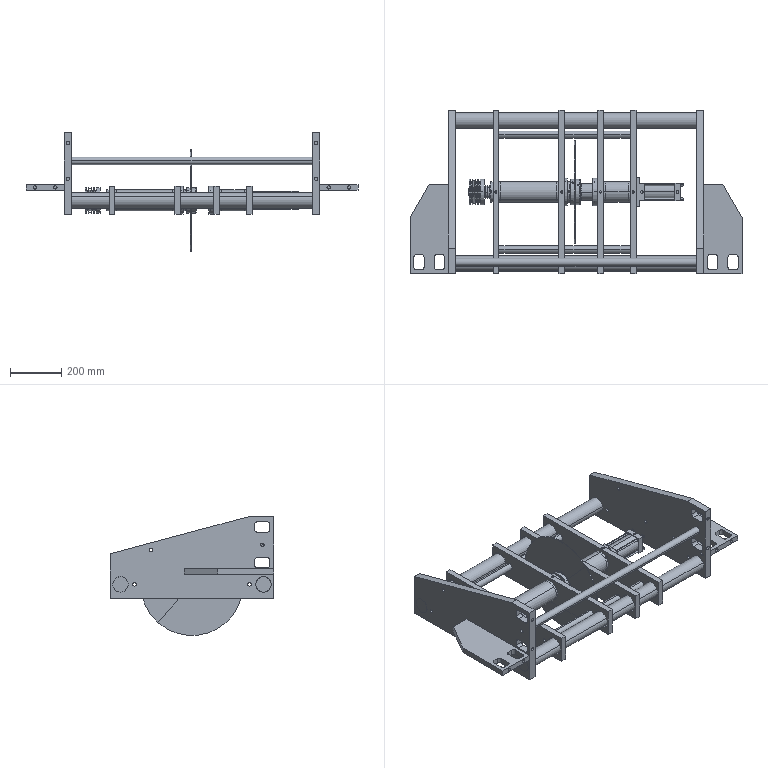Assembly | SolidWorks | mm | 50 component files | 156 solids | 2266 faces | box 1300 x 640 x 465 mm | volume 26290505 mm3 | cylinder 957 | plane 475 | sphere 364 | torus 242 | cone 228 | commonest cylinder face diameters 6.277 x72 7.03 x72 13 x64 8.017 x52 8.979 x52 20 x36 5 x34 9 x24
Bill of materials:
2-10-1WorkpieceAxisBearingHousing | 1 |  | Long hollow cylindrical tube with a wider circular flange at one end; the flange face has a large central bore, four larger through-holes and four smaller holes that look countersunk or chamfered, spaced around it.
2-10-2WorkpieceAxis | 1 |  | Long slender stepped cylindrical shaft with several diameter changes along its length; a coaxial hole with a cone-shaped bottom at one end and a small cross hole near that end.
2-10-3BearingSideCover | 2 |  | Flat circular ring-shaped plate with a large central bore, four evenly spaced through-holes near the outer edge, and a thin raised boss of smaller diameter on one face.
2-10-4Bushing | 1 |  | Thin-walled cylindrical sleeve or band with a short axial length compared to its diameter, and small chamfers on its edges.
2-10-5LockNut | 2 |  | Flat annular ring with four rectangular slots cut into its outer edge, evenly spaced; edges are chamfered.
2-10-6BearingShim | 1 |  | Thin flat annular ring (washer-like disk) with a plain round inner hole and outer edge.
2-10-7OilSealTC-40X52X7 | 2 | Rubber | Short cylindrical ring with a rectangular cross-section and an internal step or shoulder visible on one face.
2-10-8Bearing7007AC | 2 |  | Radial ball bearing-like assembly: concentric inner and outer rings with a single row of spherical balls between them, plus a thin ring-shaped element running between the balls.
2-10-9Bearing51107 | 1 |  | Axial thrust ball bearing-like assembly: two flat annular washers with a single row of balls held in a ring between them.
Flange1 | 1 |  | Thick flat circular disk with a central bore and two smaller through-holes on opposite sides; one radial hole in the outer edge; edges are chamfered.
4-12-10SplineConnectionAxisOilSealTC40X55X7 | 1 | Rubber | Cylindrical ring with a rectangular cross-section and an internal step or shoulder on one face, similar to the other stepped rings.
4-12-11TelescopicAxisOilSealTC64X80X12 | 1 | Rubber | Cylindrical ring with a fairly thin radial wall and a small internal step or groove near one face.
4-12-1ClampingTelescopicAxisHousing | 1 |  | Flanged hollow tube: a long thin-walled cylindrical sleeve with a round flange at one end that has four small holes.
4-12-2TelescopicAxis | 1 |  | Solid cylinder with a small central axial hole; looks like a thick-walled spacer or sleeve.
4-12-3ClampingAxis | 1 |  | Stepped cylindrical pin: a short larger-diameter head with a small cross hole, a raised collar, and a long, smaller-diameter shaft with a chamfered end.
4-12-4Bearing6005-2RZ | 3 |  | Ring assembly with concentric inner and outer rings and a circle of balls between them; its shape resembles a radial ball bearing.
4-12-551205Bearing | 1 |  | Axial stack of two flat annular rings with a ring of balls held between them; its shape resembles a thrust ball bearing.
4-12-6ClampingAxisBearingOuterPad | 1 |  | Short, plain, thin-walled cylindrical tube or sleeve.
4-12-7ClampingAxisBearingInnerPad | 1 |  | Plain cylindrical sleeve or bushing, with a thicker wall than the similar thin-walled tube in this set.
4-12-8ClampingAxis51205BearingShim | 1 |  | Thin flat annular ring, washer-like in shape.
4-12-9HeadlessSetScrew-D10 | 1 |  | Stepped solid round part: a smaller-diameter cylindrical spigot, a conical transition, and a larger-diameter cylindrical body with a chamfered end.
Crossbeam | 2 |  | Long, slender solid cylindrical rod with plain flat ends.
MainBracket | 2 |  | Flat plate with an irregular four-sided outline (one sloped edge), cut with two large round holes, two rounded-rectangle openings and several small holes.
SideReinforcementPlate | 2 |  | Thick flat plate with one angled corner and two rounded-rectangle through openings near one end; small holes drilled into its edge faces.
AxisHousingBracket | 4 |  | Long flat rectangular bar with three large round through-holes (one at the center, one near each end) and two small round through-holes, each just inboard of an end hole; a small hole also enters the long top edge at mid-length.
FeedingClampingCylinder | 1 |  | Cylinder-like body: a round barrel held between two square end blocks by four rods along its length, with hex nuts on the rod ends at one block. A stepped round shaft sticks out from the other end, which also has a rectangular flange with four corner holes. Each end block has a round hole in its top face.
FixedLengthRod | 1 |  | Long, slender round rod or tube with a small central hole at the end; in the end view the hole appears to have a cone-shaped, faceted bottom.
Flange2 | 1 |  | Thick ring or collar with a central through-bore, small chamfers on the outer edges, and one small radial hole in the outer cylindrical surface.
LocatingGuideBushing106 | 2 |  | Cylindrical tube or sleeve with a concentric through-bore, chamfered outer ends and chamfered bore entrances; its length is about four times its diameter.
LocatingGuideBushing130 | 2 |  | Cylindrical tube or sleeve with a concentric through-bore, chamfered outer ends and chamfered bore entrances; it is more slender than unnamed part.
LocatingGuideBushing156 | 2 |  | Long, slender cylindrical tube with a concentric through-bore, small chamfers on the outer ends and chamfered bore entrances; it is the most elongated of the similar sleeves.
Oil-impregnatedBushing | 2 |  | Thin-walled cylindrical ring or band whose width is a large fraction of its diameter, with plain inner and outer cylindrical surfaces and slight edge breaks.
SawBlade400 | 1 |  | Very thin flat circular disc with a small central hole and two smaller holes placed diagonally opposite each other near the center.
SawBladeDrivePulley | 1 |  | Multi-groove V-pulley (sheave) with four V-shaped grooves around its circumference, a wider plain cylindrical band on one side, and a central bore with a rectangular keyway.
Mates:
1. concentric | 4-12-12ClampingAxisAssembly-1/4-12-3ClampingAxis-1 face at (-152.809, -4.181, 0) dir (-1, 0, 0) r 16 | 2-10-10WorkpieceAxisAssembly-1/2-10-2WorkpieceAxis-1 face at (-157.809, -4.181, 0) dir (-1, 0, 0) r 16
2. concentric | 4-12-12ClampingAxisAssembly-1/4-12-1ClampingTelescopicAxisHousing-1 face at (-87.809, -4.181, 0) dir (-1, 0, 0) r 41 | AxisHousingBracket-1 face at (-67.809, -4.181, 0) dir (1, 0, 0) r 41
3. coincident | 4-12-12ClampingAxisAssembly-1/4-12-1ClampingTelescopicAxisHousing-1 face at (-67.809, 50.819, 0) dir (1, 0, 0) | AxisHousingBracket-1 face at (-67.809, -324.181, 55) dir (-1, 0, 0)
4. concentric | 4-12-12ClampingAxisAssembly-1/4-12-1ClampingTelescopicAxisHousing-1 face at (-87.809, 29.76, 33.941) dir (-1, 0, 0) r 3.3 | AxisHousingBracket-1 face at (-67.809, 29.76, 33.941) dir (-1, 0, 0) r 2.5
5. concentric | 2-10-10WorkpieceAxisAssembly-1/2-10-1WorkpieceAxisBearingHousing-1 face at (-187.809, -4.181, 0) dir (1, 0, 0) r 41 | AxisHousingBracket-2 face at (60.191, -4.181, 0) dir (1, 0, 0) r 41
6. concentric | AxisHousingBracket-1 face at (-67.809, 275.819, 0) dir (1, 0, 0) r 35 | AxisHousingBracket-2 face at (60.191, 275.819, 0) dir (1, 0, 0) r 35
7. coincident | 4-12-12ClampingAxisAssembly-1/4-12-1ClampingTelescopicAxisHousing-1 face at (82.191, 36.819, 0) dir (1, 0, 0) | AxisHousingBracket-2 face at (82.191, -324.181, 55) dir (1, 0, 0)
8. concentric | 2-10-10WorkpieceAxisAssembly-1/2-10-1WorkpieceAxisBearingHousing-1 face at (-187.809, -4.181, 0) dir (1, 0, 0) r 41 | AxisHousingBracket-3 face at (-197.809, -4.181, 0) dir (-1, 0, 0) r 41
9. coincident | 2-10-10WorkpieceAxisAssembly-1/2-10-1WorkpieceAxisBearingHousing-1 face at (-197.809, 36.556, 36.952) dir (-1, 0, 0) | AxisHousingBracket-3 face at (-197.809, 315.819, 55) dir (1, 0, 0)
10. coincident | AxisHousingBracket-1 face at (-67.809, 315.819, 55) dir (0, 0, 1) | AxisHousingBracket-3 face at (-197.809, -324.181, 55) dir (0, 0, 1)
11. concentric | 2-10-10WorkpieceAxisAssembly-1/2-10-1WorkpieceAxisBearingHousing-1 face at (-187.809, -4.181, 0) dir (1, 0, 0) r 41 | AxisHousingBracket-4 face at (-477.809, -4.181, 0) dir (1, 0, 0) r 41
12. parallel | AxisHousingBracket-3 face at (-197.809, -324.181, 55) dir (0, 0, 1) | AxisHousingBracket-4 face at (-477.809, 315.819, 55) dir (0, 0, 1)
13. coincident | 2-10-10WorkpieceAxisAssembly-1/2-10-3BearingSideCover-2 edge at (-477.809, -4.181, 0) dir (1, 0, 0) r 41 | AxisHousingBracket-4 face at (-477.809, -324.181, 55) dir (-1, 0, 0)
14. distance | AxisHousingBracket-1 face at (-67.809, -324.181, 55) dir (-1, 0, 0) | AxisHousingBracket-3 face at (-197.809, 315.819, 55) dir (1, 0, 0)
15. coincident | AxisHousingBracket-3 face at (-197.809, 315.819, 55) dir (1, 0, 0) | LocatingGuideBushing130-1 face at (-197.809, -229.181, 0) dir (-1, 0, 0)
16. concentric | AxisHousingBracket-3 face at (-219.809, -229.181, 0) dir (1, 0, 0) r 6.5 | LocatingGuideBushing130-1 face at (-67.809, -229.181, 0) dir (-1, 0, 0) r 14
17. coincident | AxisHousingBracket-3 face at (-197.809, 315.819, 55) dir (1, 0, 0) | LocatingGuideBushing130-2 face at (-197.809, 220.819, 0) dir (-1, 0, 0)
18. concentric | AxisHousingBracket-3 face at (-219.809, 220.819, 0) dir (1, 0, 0) r 6.5 | LocatingGuideBushing130-2 face at (-67.809, 220.819, 0) dir (-1, 0, 0) r 6.5
19. concentric | LocatingGuideBushing130-2 face at (-67.809, 220.819, 0) dir (-1, 0, 0) r 14 | LocatingGuideBushing106-1 face at (-45.809, 220.819, 0) dir (1, 0, 0) r 14
20. coincident | AxisHousingBracket-2 face at (60.191, -324.181, 55) dir (-1, 0, 0) | LocatingGuideBushing106-1 face at (60.191, 220.819, 0) dir (1, 0, 0)
21. concentric | AxisHousingBracket-3 face at (-219.809, 220.819, 0) dir (1, 0, 0) r 6.5 | LocatingGuideBushing156-1 face at (-219.809, 220.819, 0) dir (-1, 0, 0) r 14
22. coincident | AxisHousingBracket-3 face at (-219.809, 315.819, 55) dir (-1, 0, 0) | LocatingGuideBushing156-1 face at (-219.809, 220.819, 0) dir (1, 0, 0)
23. concentric | AxisHousingBracket-3 edge at (-219.809, -229.181, 0) dir (1, 0, 0) r 6.5 | LocatingGuideBushing156-2 face at (-219.809, -229.181, 0) dir (-1, 0, 0) r 14
24. coincident | AxisHousingBracket-3 face at (-219.809, 315.819, 55) dir (-1, 0, 0) | LocatingGuideBushing156-2 face at (-219.809, -229.181, 0) dir (1, 0, 0)
25. concentric | AxisHousingBracket-1 face at (-45.809, -229.181, 0) dir (-1, 0, 0) r 6.5 | LocatingGuideBushing106-2 face at (-45.809, -229.181, 0) dir (1, 0, 0) r 14
26. coincident | AxisHousingBracket-2 face at (60.191, -324.181, 55) dir (-1, 0, 0) | LocatingGuideBushing106-2 face at (60.191, -229.181, 0) dir (1, 0, 0)
27. concentric | AxisHousingBracket-4 face at (-477.809, 275.819, 0) dir (1, 0, 0) r 35 | Oil-impregnatedBushing-1 face at (-455.809, 275.819, 0) dir (-1, 0, 0) r 30
28. coincident | AxisHousingBracket-4 face at (-477.809, -324.181, 55) dir (-1, 0, 0) | Oil-impregnatedBushing-1 face at (-477.809, 275.819, 0) dir (-1, 0, 0)
29. concentric | AxisHousingBracket-3 face at (-197.809, 275.819, 0) dir (-1, 0, 0) r 35 | Oil-impregnatedBushing-2 face at (-219.809, 275.819, 0) dir (1, 0, 0) r 30
30. coincident | AxisHousingBracket-3 face at (-197.809, 315.819, 55) dir (1, 0, 0) | Oil-impregnatedBushing-2 face at (-197.809, 275.819, 0) dir (1, 0, 0)
31. concentric | 2-10-10WorkpieceAxisAssembly-1/2-10-2WorkpieceAxis-1 face at (-157.809, -4.181, 0) dir (-1, 0, 0) r 16 | SawBlade400-1 face at (-159.809, -4.181, 0) dir (1, 0, 0) r 16
32. concentric | 4-12-12ClampingAxisAssembly-1/4-12-1ClampingTelescopicAxisHousing-1 face at (-87.809, -4.181, 0) dir (-1, 0, 0) r 32 | FeedingClampingCylinder-1 face at (74.191, -4.181, 0) dir (1, 0, 0) r 12.5
33. coincident | AxisHousingBracket-2 face at (82.191, -324.181, 55) dir (1, 0, 0) | FeedingClampingCylinder-1 face at (82.191, 23.819, -28) dir (-1, 0, 0)
34. concentric | 2-10-10WorkpieceAxisAssembly-1/2-10-2WorkpieceAxis-1 face at (-436.912, -4.181, 0) dir (-1, 0, 0) r 15 | SawBladeDrivePulley-2 face at (-617.309, -4.181, 0) dir (-1, 0, 0) r 15
35. coincident | 2-10-10WorkpieceAxisAssembly-1/Flange1-1 face at (-159.809, -4.181, 0) dir (1, 0, 0) | SawBlade400-1 face at (-159.809, -4.181, 0) dir (-1, 0, 0)
36. concentric | 2-10-10WorkpieceAxisAssembly-1/Flange1-1 face at (-173.809, 16.982, -23.331) dir (1, 0, 0) r 5 | SawBlade400-1 face at (-159.809, 16.982, -23.331) dir (1, 0, 0) r 5.5
37. concentric | 4-12-12ClampingAxisAssembly-1/4-12-3ClampingAxis-1 face at (-152.809, -4.181, 0) dir (-1, 0, 0) r 16 | Flange2-1 face at (-156.809, -4.181, 0) dir (1, 0, 0) r 16
38. coincident | 4-12-12ClampingAxisAssembly-1/4-12-3ClampingAxis-1 face at (-136.809, 4.607, 13.371) dir (-1, 0, 0) | Flange2-1 face at (-136.809, -4.181, 0) dir (1, 0, 0)
39. concentric | 4-12-12ClampingAxisAssembly-1/4-12-3ClampingAxis-1 face at (-144.809, 1.311, 8.357) dir (0, 0.5492, 0.8357) r 3 | Flange2-1 face at (-144.809, 23.281, 41.783) dir (0, 0.5492, 0.8357) r 3.4
40. concentric | Assembly2-1/Crossbeam-1 face at (346.98, 275.819, 0) dir (-1, 0, 0) r 30 | AxisHousingBracket-2 face at (60.191, 275.819, 0) dir (1, 0, 0) r 35
41. concentric | Assembly2-1/Crossbeam-2 face at (346.98, -284.181, 0) dir (-1, 0, 0) r 30 | AxisHousingBracket-2 face at (60.191, -284.181, 0) dir (1, 0, 0) r 35
42. concentric | Assembly2-1/MainBracket-1 face at (-625.02, -279.181, 155) dir (-1, 0, 0) r 7 | FixedLengthRod-1 face at (-625.02, -279.181, 155) dir (1, 0, 0) r 15
43. coincident | Assembly2-1/MainBracket-1 face at (-625.02, -324.181, 55) dir (1, 0, 0) | FixedLengthRod-1 face at (-625.02, -279.181, 155) dir (-1, 0, 0)
44. concentric | 2-10-1WorkpieceAxisBearingHousing-1 face at (-124.268, 52.47, 0) dir (-1, 0, 0) r 40.9 | 2-10-2WorkpieceAxis-1 face at (-154.268, 52.47, 0) dir (1, 0, 0) r 17.4
45. coincident | 2-10-1WorkpieceAxisBearingHousing-1 face at (-124.268, 83.47, 0) dir (-1, 0, 0) | 2-10-3BearingSideCover-1 face at (-124.268, 81.461, -28.991) dir (1, 0, 0)
46. concentric | 2-10-1WorkpieceAxisBearingHousing-1 face at (-124.268, 77.926, 25.456) dir (-1, 0, 0) r 2.1 | 2-10-3BearingSideCover-1 face at (-135.268, 77.926, 25.456) dir (-1, 0, 0) r 4.5
47. concentric | 2-10-2WorkpieceAxis-1 face at (-154.268, 52.47, 0) dir (1, 0, 0) r 17.4 | 2-10-3BearingSideCover-1 face at (-110.214, 52.47, 0) dir (1, 0, 0) r 41
48. concentric | 2-10-1WorkpieceAxisBearingHousing-1 face at (-124.268, 52.47, 0) dir (-1, 0, 0) r 31 | 2-10-3BearingSideCover-2 face at (151.679, 52.47, 0) dir (-1, 0, 0) r 20.5
49. coincident | 2-10-1WorkpieceAxisBearingHousing-1 face at (165.732, 83.47, 0) dir (1, 0, 0) | 2-10-3BearingSideCover-2 face at (165.732, 81.461, 28.991) dir (-1, 0, 0)
50. concentric | 2-10-1WorkpieceAxisBearingHousing-1 face at (165.732, 77.926, 25.456) dir (1, 0, 0) r 2.1 | 2-10-3BearingSideCover-2 face at (176.732, 77.926, 25.456) dir (1, 0, 0) r 2.75
51. concentric | 2-10-2WorkpieceAxis-1 face at (-154.268, 52.47, 0) dir (1, 0, 0) r 17.5 | 2-10-4Bushing-1 face at (178.732, 52.47, 0) dir (-1, 0, 0) r 17.5
52. concentric | 2-10-2WorkpieceAxis-1 face at (-154.268, 52.47, 0) dir (1, 0, 0) r 17.5 | 2-10-5LockNut-1 face at (186.732, 52.47, 0) dir (-1, 0, 0) r 17.5
53. concentric | 2-10-2WorkpieceAxis-1 face at (-154.268, 52.47, 0) dir (1, 0, 0) r 17.5 | 2-10-5LockNut-2 face at (178.732, 52.47, 0) dir (-1, 0, 0) r 17.5
54. coincident | 2-10-5LockNut-1 face at (186.732, 52.47, 0) dir (-1, 0, 0) | 2-10-5LockNut-2 face at (186.732, 52.47, 0) dir (1, 0, 0)
55. coincident | 2-10-4Bushing-1 face at (178.732, 52.47, 0) dir (1, 0, 0) | 2-10-5LockNut-2 face at (178.732, 52.47, 0) dir (-1, 0, 0)
56. concentric | 2-10-2WorkpieceAxis-1 face at (-154.268, 52.47, 0) dir (1, 0, 0) r 17.5 | 2-10-6BearingShim-1 face at (-106.268, 52.47, 0) dir (-1, 0, 0) r 17.75
57. concentric | 2-10-3BearingSideCover-2 face at (151.679, 52.47, 0) dir (-1, 0, 0) r 27.5 | 2-10-7OilSealTC-40X52X7-1 face at (164.732, 52.47, 0) dir (1, 0, 0) r 20
58. coincident | 2-10-3BearingSideCover-2 face at (171.732, 71.915, 19.445) dir (-1, 0, 0) | 2-10-7OilSealTC-40X52X7-1 face at (171.732, 52.47, 0) dir (1, 0, 0)
59. concentric | 2-10-2WorkpieceAxis-1 face at (-154.268, 52.47, 0) dir (1, 0, 0) r 17.5 | 2-10-7OilSealTC-40X52X7-2 face at (-123.268, 52.47, 0) dir (-1, 0, 0) r 27.5
60. coincident | 2-10-3BearingSideCover-1 face at (-130.268, 71.915, -19.445) dir (1, 0, 0) | 2-10-7OilSealTC-40X52X7-2 face at (-130.268, 52.47, 0) dir (-1, 0, 0)
61. concentric | 2-10-2WorkpieceAxis-1 face at (-154.268, 52.47, 0) dir (1, 0, 0) r 17.4 | 2-10-8Bearing7007AC-1 face at (-175.268, 52.47, 0) dir (-1, 0, 0) r 17.5
62. coincident | 2-10-6BearingShim-1 face at (-108.268, 52.47, 0) dir (-1, 0, 0) | 2-10-8Bearing7007AC-1 face at (-108.268, 35.095, -2.092) dir (1, 0, 0)
63. coincident | 2-10-6BearingShim-1 face at (-106.268, 52.47, 0) dir (1, 0, 0) | 2-10-9Bearing51107-1 face at (-106.268, 73.433, 15.38) dir (-1, 0, 0)
64. concentric | 2-10-2WorkpieceAxis-1 face at (-154.268, 52.47, 0) dir (1, 0, 0) r 17.5 | 2-10-9Bearing51107-1 face at (-158.268, 52.47, 0) dir (-1, 0, 0) r 18.5
65. concentric | 2-10-2WorkpieceAxis-1 face at (-154.268, 52.47, 0) dir (1, 0, 0) r 17.5 | 2-10-8Bearing7007AC-2 face at (216.732, 52.47, 0) dir (1, 0, 0) r 17.5
66. coincident | 2-10-4Bushing-1 face at (163.732, 52.47, 0) dir (-1, 0, 0) | 2-10-8Bearing7007AC-2 face at (163.732, 52.323, 17.499) dir (1, 0, 0)
67. coincident | 2-10-1WorkpieceAxisBearingHousing-1 face at (149.732, 74.97, 0) dir (1, 0, 0) | 2-10-8Bearing7007AC-2 face at (149.732, 60.101, 25.739) dir (-1, 0, 0)
68. coincident | 2-10-1WorkpieceAxisBearingHousing-1 face at (-94.268, 78.47, 0) dir (-1, 0, 0) | 2-10-9Bearing51107-1 face at (-94.268, 65.942, 22.237) dir (1, 0, 0)
69. coincident | 2-10-2WorkpieceAxis-1 face at (-122.268, 71.989, 4.357) dir (1, 0, 0) | 2-10-8Bearing7007AC-1 face at (-122.268, 35.095, -2.092) dir (-1, 0, 0)
70. concentric | 2-10-2WorkpieceAxis-1 face at (-154.268, 52.47, 0) dir (1, 0, 0) r 16 | Flange1-1 face at (-138.268, 52.47, 0) dir (-1, 0, 0) r 16
71. coincident | 2-10-2WorkpieceAxis-1 face at (-138.268, 68.085, 3.486) dir (-1, 0, 0) | Flange1-1 face at (-138.268, 52.47, 0) dir (1, 0, 0)
72. concentric | 4-12-1ClampingTelescopicAxisHousing-1 face at (-32.244, 37.13, 0) dir (-1, 0, 0) r 32 | 4-12-2TelescopicAxis-1 face at (-77.244, 37.13, 0) dir (-1, 0, 0) r 32
73. tangent | 4-12-1ClampingTelescopicAxisHousing-1 face at (35.756, 37.13, 0) dir (0, -1, 0) r 4.25 | 4-12-2TelescopicAxis-1 edge at (58.756, 68.847, 4.25) dir (-1, 0, 0)
74. concentric | 4-12-2TelescopicAxis-1 face at (-77.244, 37.13, 0) dir (-1, 0, 0) r 23.5 | 4-12-3ClampingAxis-1 face at (-97.244, 37.13, 0) dir (-1, 0, 0) r 20
75. concentric | 4-12-2TelescopicAxis-1 face at (-77.244, 37.13, 0) dir (-1, 0, 0) r 27.5 | 4-12-10SplineConnectionAxisOilSealTC40X55X7-1 face at (-70.244, 37.13, 0) dir (-1, 0, 0) r 27.5
76. coincident | 4-12-2TelescopicAxis-1 face at (-70.244, 37.315, -23.499) dir (-1, 0, 0) | 4-12-10SplineConnectionAxisOilSealTC40X55X7-1 face at (-70.244, 37.13, 0) dir (1, 0, 0)
77. concentric | 4-12-2TelescopicAxis-1 face at (-77.244, 37.13, 0) dir (-1, 0, 0) r 23.5 | 4-12-4Bearing6005-2RZ-1 face at (7.756, 37.13, 0) dir (1, 0, 0) r 12.5
78. concentric | 4-12-2TelescopicAxis-1 face at (-77.244, 37.13, 0) dir (-1, 0, 0) r 23.5 | 4-12-4Bearing6005-2RZ-3 face at (-4.244, 37.13, 0) dir (1, 0, 0) r 12.5
79. concentric | 4-12-2TelescopicAxis-1 face at (-77.244, 37.13, 0) dir (-1, 0, 0) r 23.5 | 4-12-4Bearing6005-2RZ-2 face at (-66.244, 37.13, 0) dir (-1, 0, 0) r 12.5
80. concentric | 4-12-2TelescopicAxis-1 face at (-77.244, 37.13, 0) dir (-1, 0, 0) r 32 | 4-12-551205Bearing-1 face at (-48.244, 37.13, 0) dir (-1, 0, 0) r 13.5
81. concentric | 4-12-2TelescopicAxis-1 face at (-77.244, 37.13, 0) dir (-1, 0, 0) r 23.5 | 4-12-8ClampingAxis51205BearingShim-1 face at (-0.2436, 37.13, 0) dir (1, 0, 0) r 12.5
82. coincident | 4-12-551205Bearing-1 face at (1.756, 23.854, 19.39) dir (-1, 0, 0) | 4-12-8ClampingAxis51205BearingShim-1 face at (1.756, 37.13, 0) dir (1, 0, 0)
83. coincident | 4-12-4Bearing6005-2RZ-2 face at (-0.2436, 24.996, 3) dir (1, 0, 0) | 4-12-8ClampingAxis51205BearingShim-1 face at (-0.2436, 37.13, 0) dir (-1, 0, 0)
84. concentric | 4-12-3ClampingAxis-1 face at (-97.244, 37.13, 0) dir (-1, 0, 0) r 12.5 | 4-12-6ClampingAxisBearingOuterPad-1 face at (-46.244, 37.13, 0) dir (1, 0, 0) r 19.5
85. concentric | 4-12-3ClampingAxis-1 face at (-97.244, 37.13, 0) dir (-1, 0, 0) r 12.5 | 4-12-7ClampingAxisBearingInnerPad-1 face at (-46.244, 37.13, 0) dir (1, 0, 0) r 12.5
86. coincident | 4-12-4Bearing6005-2RZ-1 face at (-46.244, 44.486, 18.722) dir (1, 0, 0) | 4-12-6ClampingAxisBearingOuterPad-1 face at (-46.244, 37.13, 0) dir (-1, 0, 0)
87. coincident | 4-12-4Bearing6005-2RZ-1 face at (-46.244, 38.101, 12.462) dir (1, 0, 0) | 4-12-7ClampingAxisBearingInnerPad-1 face at (-46.244, 37.13, 0) dir (-1, 0, 0)
88. coincident | 4-12-4Bearing6005-2RZ-1 face at (-58.244, 38.101, 12.462) dir (-1, 0, 0) | 4-12-4Bearing6005-2RZ-3 face at (-58.244, 49.084, 3.654) dir (1, 0, 0)
89. coincident | 4-12-4Bearing6005-2RZ-2 face at (-12.244, 24.996, 3) dir (-1, 0, 0) | 4-12-7ClampingAxisBearingInnerPad-1 face at (-12.244, 37.13, 0) dir (1, 0, 0)
90. coincident | 4-12-2TelescopicAxis-1 face at (16.756, 37.248, -15) dir (-1, 0, 0) | 4-12-551205Bearing-1 face at (16.756, 17.438, 12.825) dir (1, 0, 0)
91. concentric | 4-12-2TelescopicAxis-1 face at (-77.244, 37.13, 0) dir (-1, 0, 0) r 32 | 4-12-11TelescopicAxisOilSealTC64X80X12-1 face at (-20.244, 37.13, 0) dir (-1, 0, 0) r 32
92. coincident | 4-12-1ClampingTelescopicAxisHousing-1 face at (-20.244, 69.13, 0) dir (-1, 0, 0) | 4-12-11TelescopicAxisOilSealTC64X80X12-1 face at (-20.244, 37.13, 0) dir (1, 0, 0)
93. distance | 4-12-1ClampingTelescopicAxisHousing-1 face at (137.756, 78.13, 0) dir (1, 0, 0) | 4-12-2TelescopicAxis-1 face at (77.756, 37.382, -31.999) dir (1, 0, 0)
94. coincident | 4-12-3ClampingAxis-1 face at (-70.244, 48.115, 16.713) dir (1, 0, 0) | 4-12-4Bearing6005-2RZ-3 face at (-70.244, 49.084, 3.654) dir (-1, 0, 0)
95. concentric | 4-12-1ClampingTelescopicAxisHousing-1 face at (35.756, 37.13, 0) dir (0, -1, 0) r 4.25 | 4-12-9HeadlessSetScrew-D10-1 face at (35.756, 77.161, 0) dir (0, 1, 0) r 3.5
96. distance | 4-12-2TelescopicAxis-1 vertex at (-3.244, 65.161, -3.779) dir (1, 0, 0) | 4-12-9HeadlessSetScrew-D10-1 face at (35.756, 67.161, 0) dir (0, -1, 0)
97. concentric | MainBracket-1 face at (-607.023, 275.819, 0) dir (1, 0, 0) r 30 | Crossbeam-1 face at (392.977, 275.819, 0) dir (-1, 0, 0) r 30
98. coincident | MainBracket-1 face at (-607.023, -324.181, 55) dir (-1, 0, 0) | Crossbeam-1 face at (-607.023, 275.819, 0) dir (-1, 0, 0)
99. coincident | MainBracket-2 face at (392.977, -324.181, 55) dir (1, 0, 0) | Crossbeam-1 face at (392.977, 275.819, 0) dir (1, 0, 0)
100. concentric | MainBracket-1 face at (-607.023, -284.181, 0) dir (1, 0, 0) r 30 | Crossbeam-2 face at (392.977, -284.181, 0) dir (-1, 0, 0) r 30
101. coincident | MainBracket-1 face at (-607.023, -324.181, 55) dir (-1, 0, 0) | Crossbeam-2 face at (-607.023, -284.181, 0) dir (-1, 0, 0)
102. coincident | MainBracket-1 face at (-607.023, -324.181, 55) dir (-1, 0, 0) | SideReinforcementPlate-1 face at (-607.023, 25.819, 62) dir (1, 0, 0)
103. distance | MainBracket-1 face at (-607.023, 315.819, -55) dir (0, 0, -1) | SideReinforcementPlate-1 face at (-607.023, -324.181, 40) dir (0, 0, -1)
104. coincident | MainBracket-1 face at (-607.023, -324.181, -55) dir (0, -1, 0) | SideReinforcementPlate-1 face at (-607.023, -324.181, 62) dir (0, -1, 0)
105. coincident | MainBracket-2 face at (392.977, -324.181, 55) dir (1, 0, 0) | SideReinforcementPlate-3 face at (392.977, 25.819, 40) dir (-1, 0, 0)
106. distance | MainBracket-2 face at (364.977, 315.819, -55) dir (0, 0, -1) | SideReinforcementPlate-3 face at (392.977, -324.181, 40) dir (0, 0, -1)
107. coincident | MainBracket-2 face at (364.977, -324.181, -55) dir (0, -1, 0) | SideReinforcementPlate-3 face at (392.977, -324.181, 40) dir (0, -1, 0)